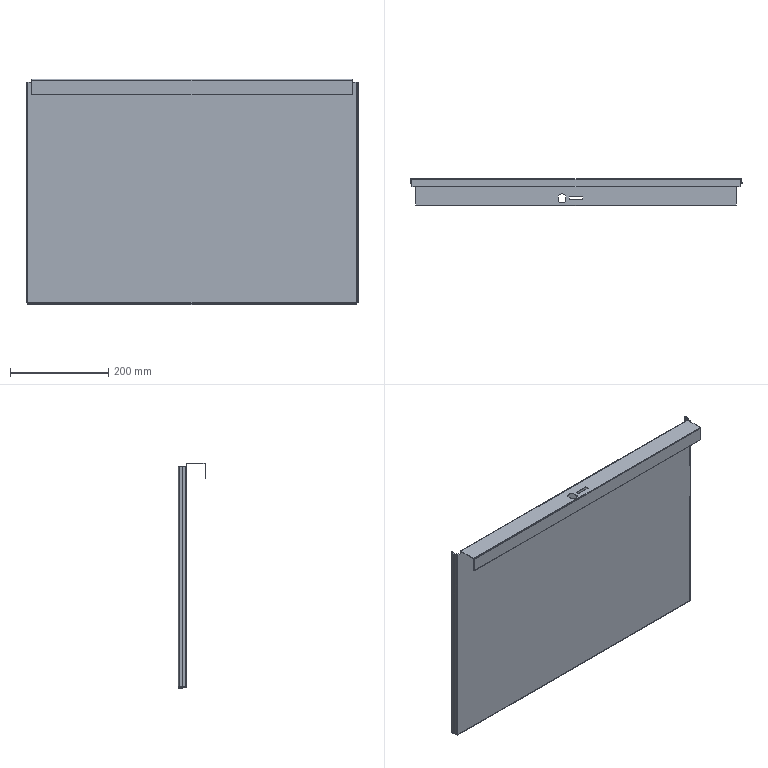Component | SolidWorks | PC-CAJ-P08-1_PM-CAJ-P35-1 | 1 solid | 82 faces | volume 388209 mm3 | plane 64 | cylinder 18 | commonest cylinder face diameters 3 x5 1 x5 1.3 x3 3.3 x3 18.708 x2 | material Plain Carbon Steel